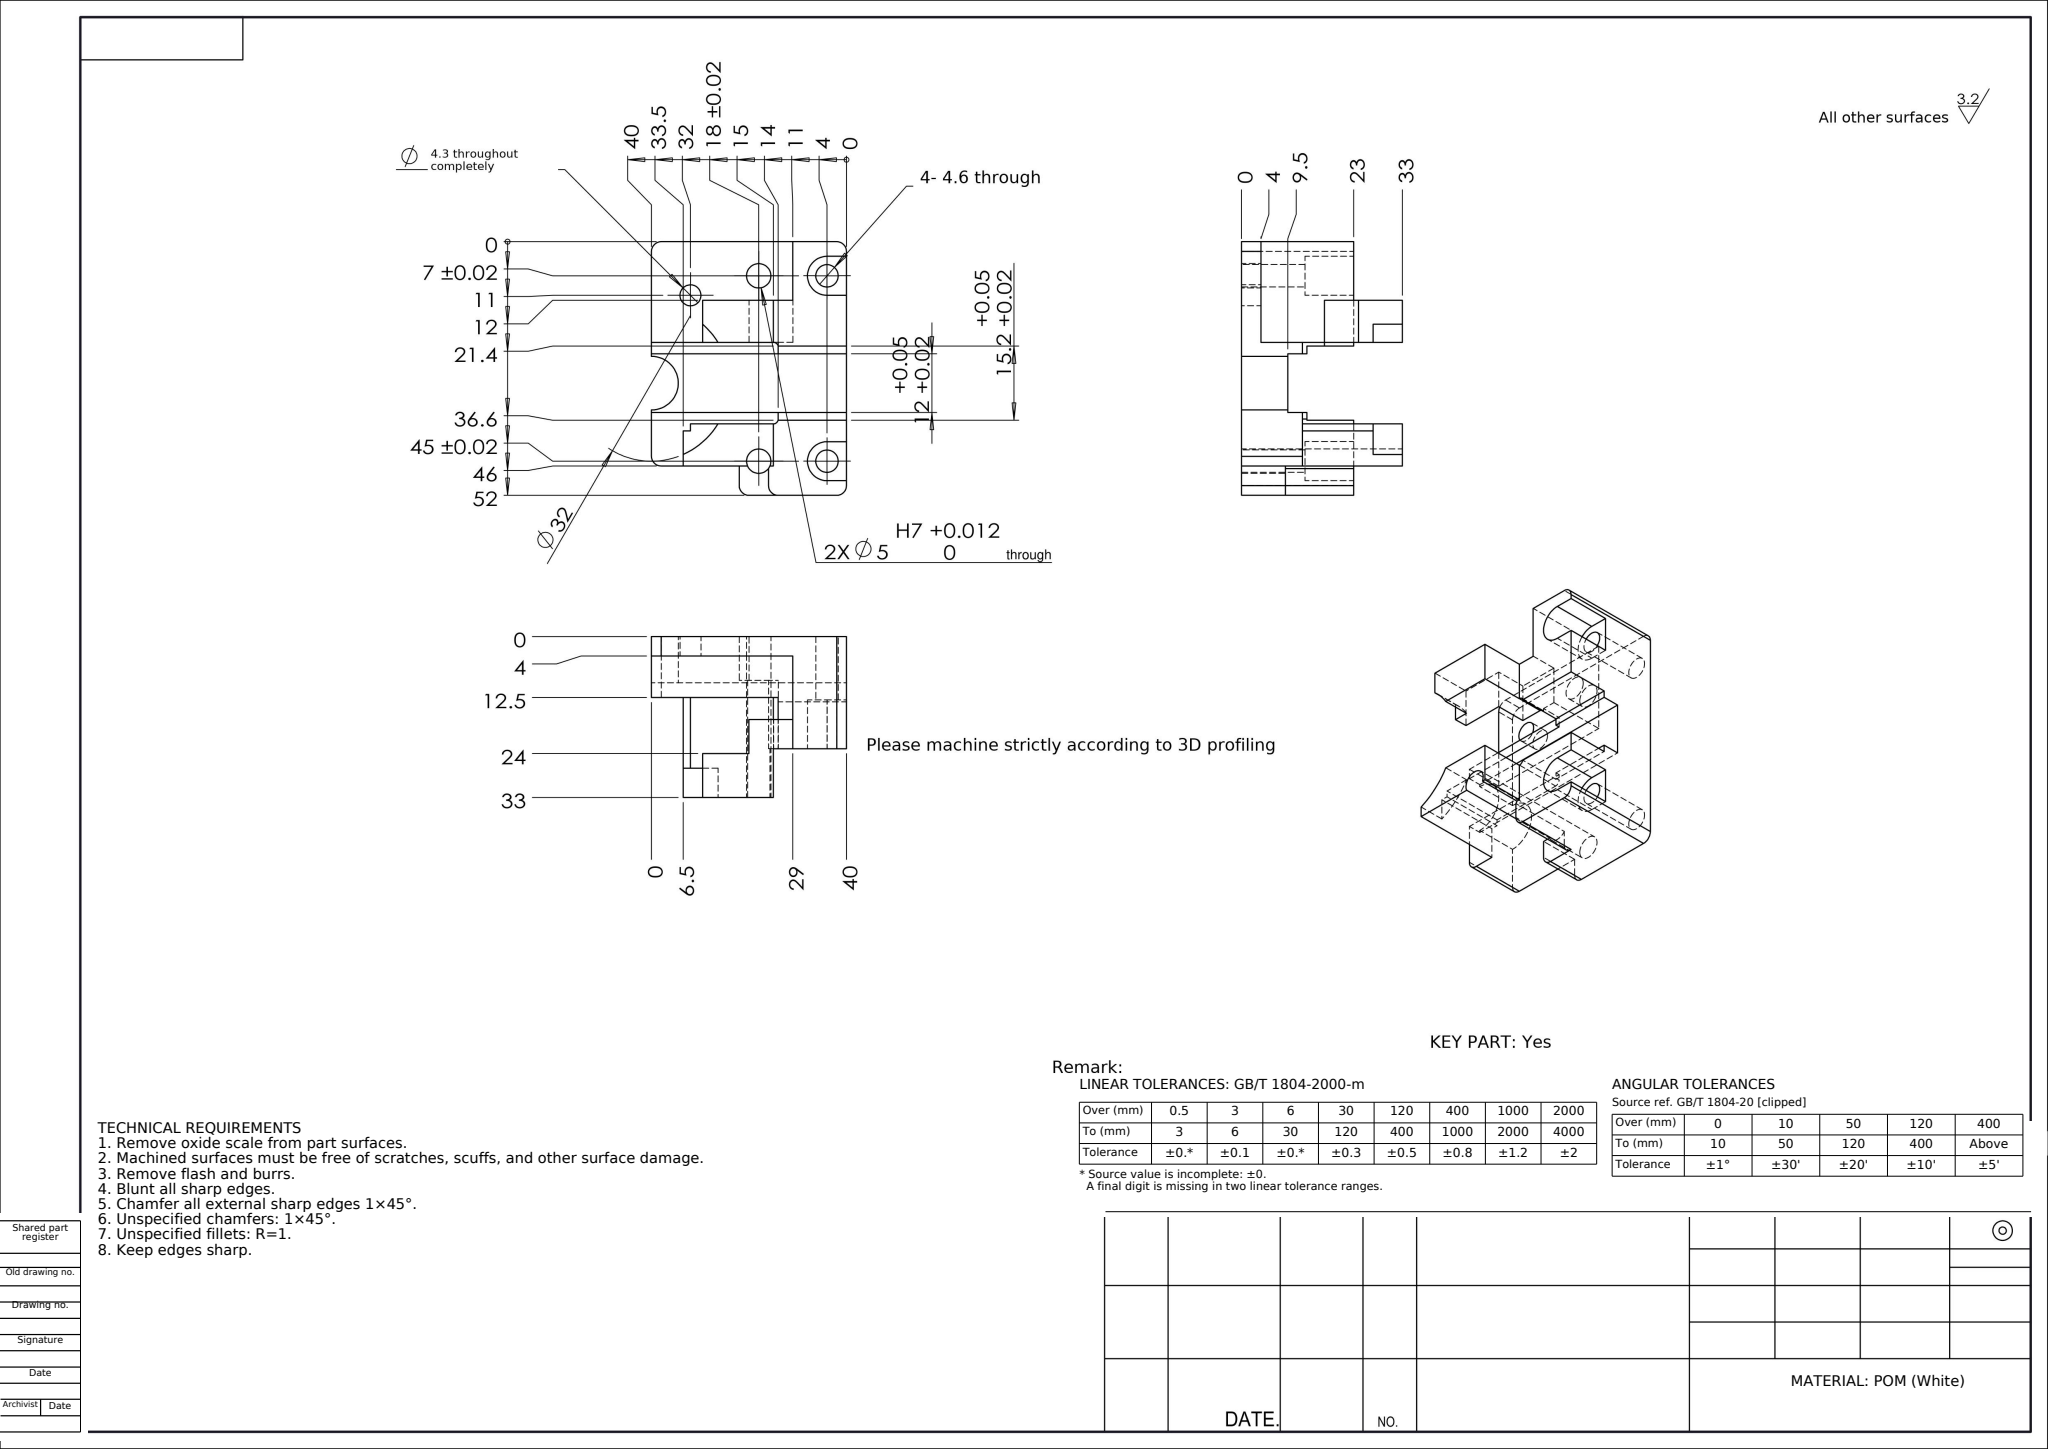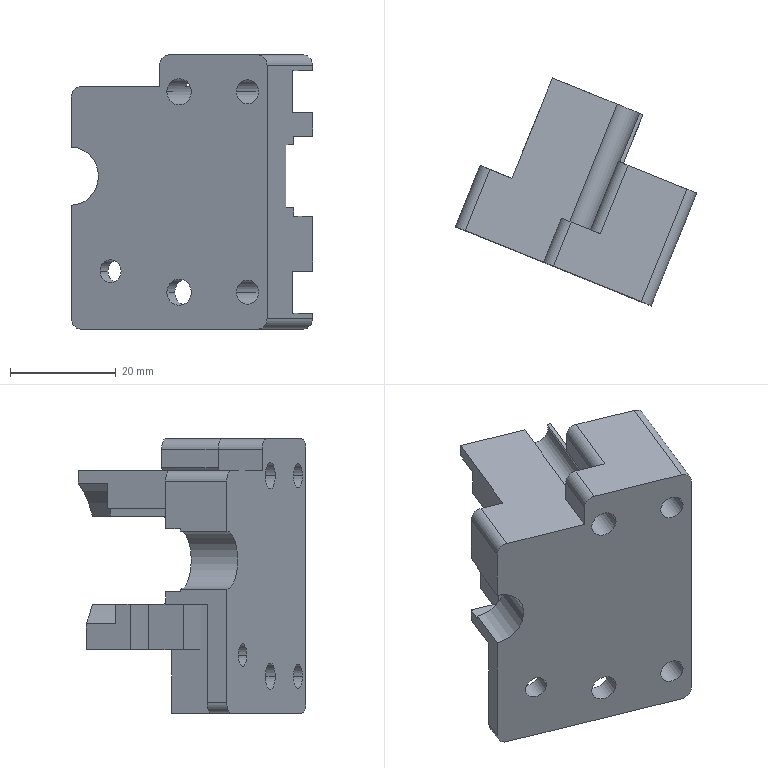Part | SolidWorks | mm | material POM (White) | 1 solid | 74 faces | box 45.7 x 43.15 x 52 mm | volume 24934 mm3 | plane 49 | cylinder 25 | commonest cylinder face diameters 4 x6 5 x4 4.6 x4 8 x4 4.3 x2 32 x2 2 x2 11 x1